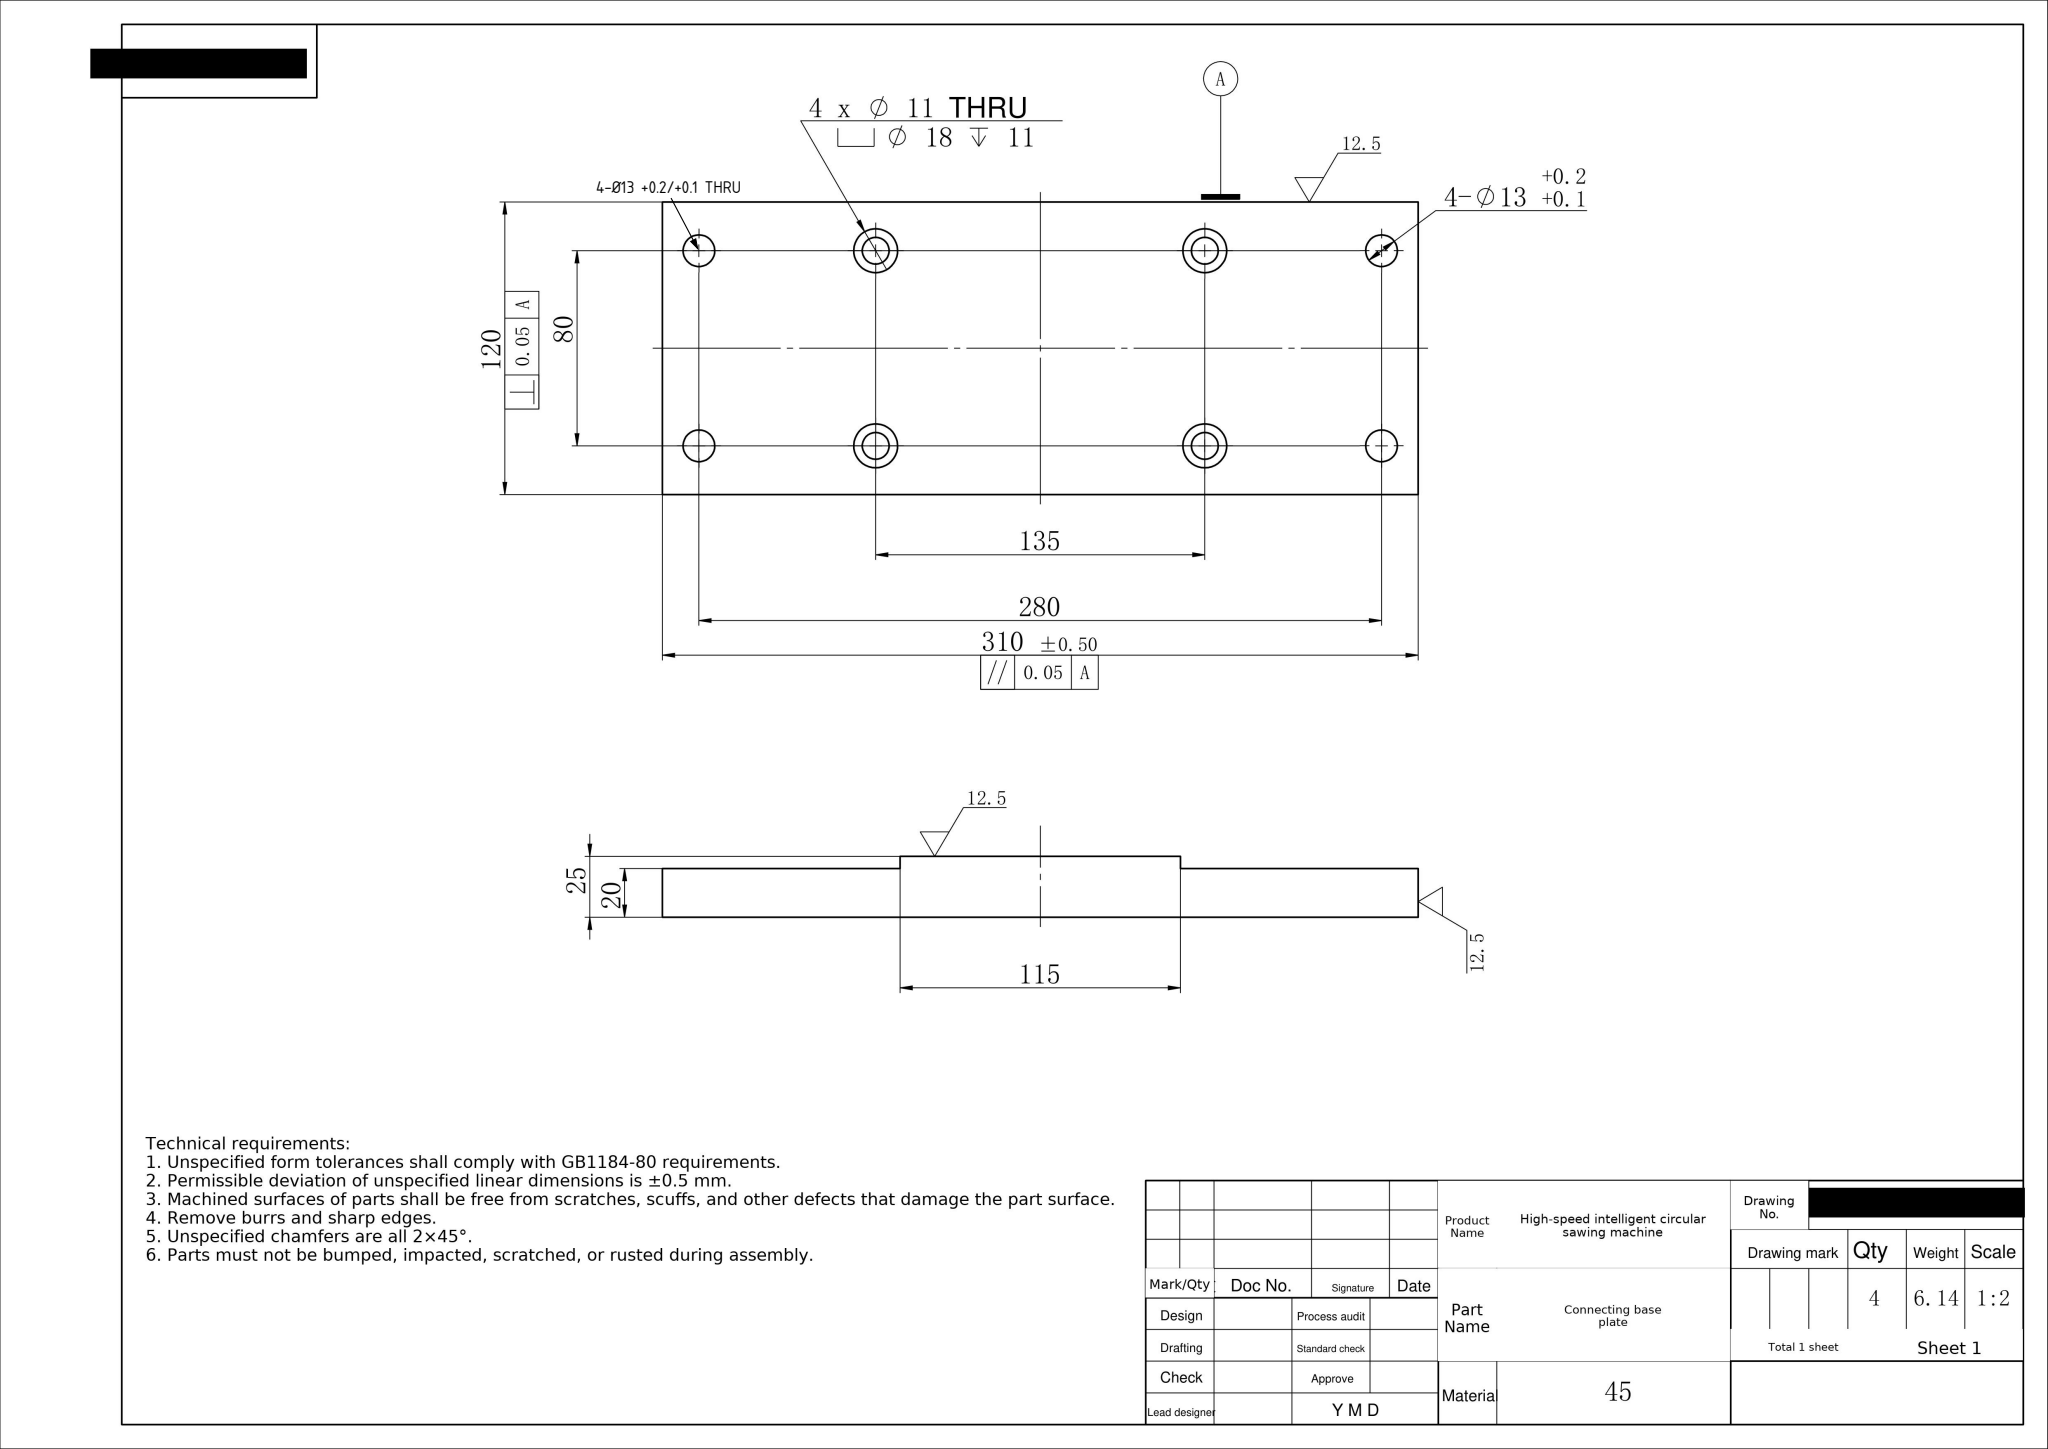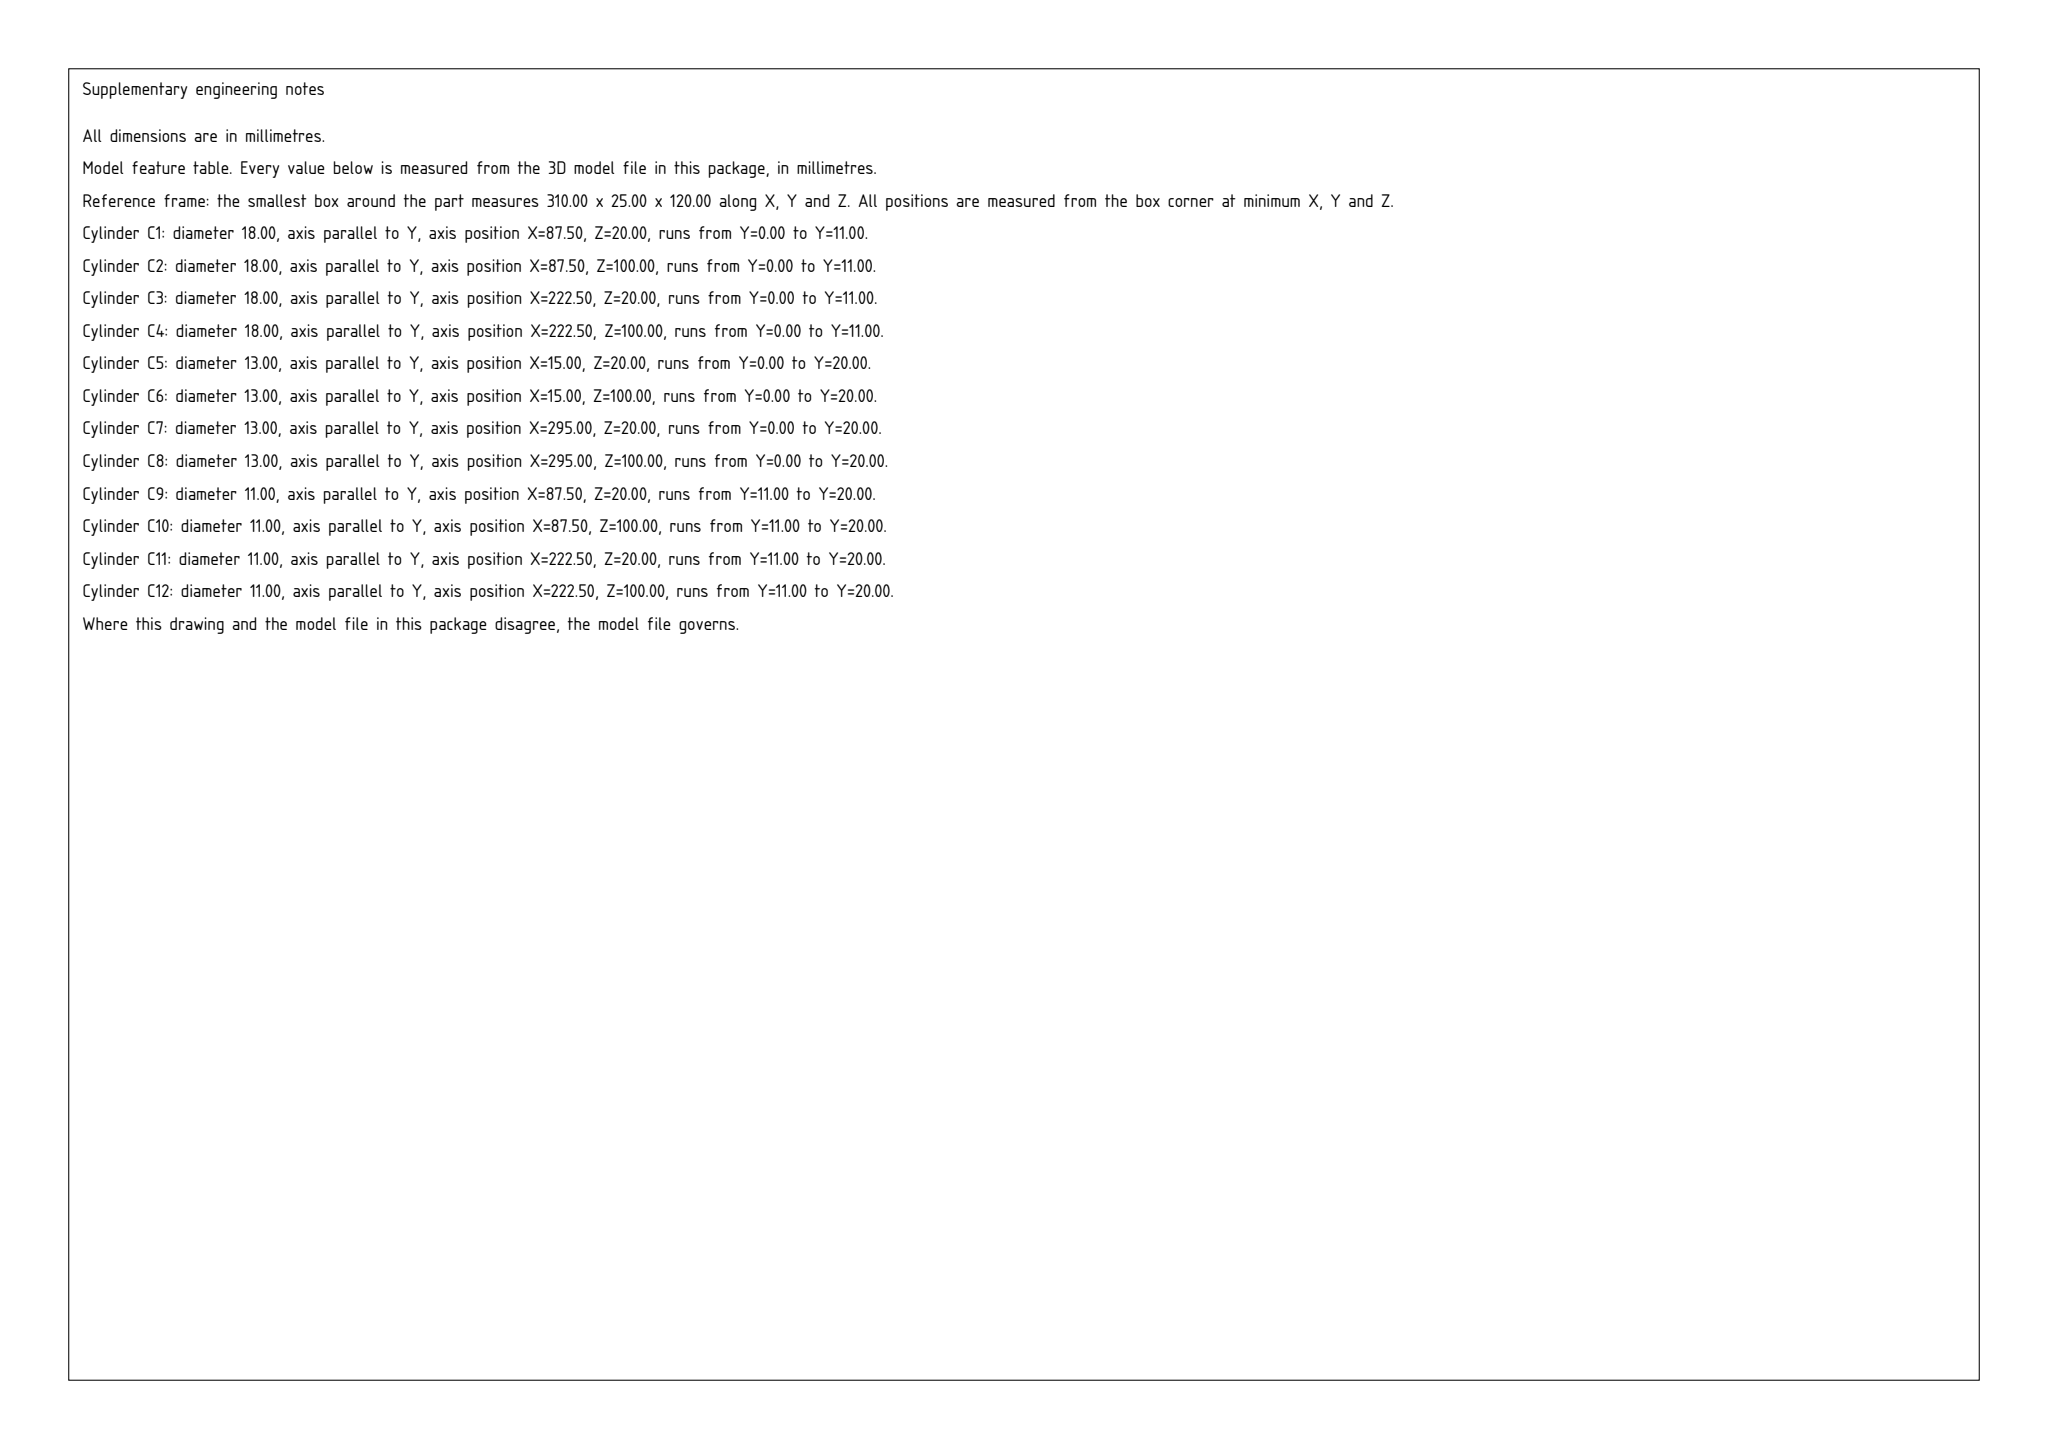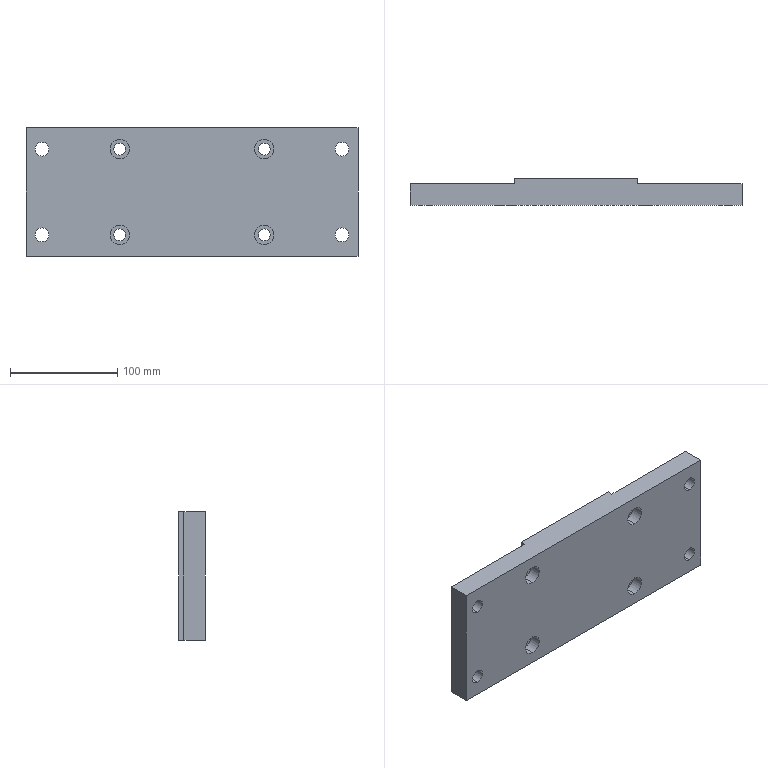Part | SolidWorks | mm | material 45 | 1 solid | 38 faces | box 310 x 25 x 120 mm | volume 787764 mm3 | cylinder 24 | plane 14 | commonest cylinder face diameters 18 x8 11 x8 13 x8
Drawing notes:
4-Ø13 +0.2/+0.1 THRU 20 THK END SECTIONS | from the solid: Ø13 cylinders, axis y, length 20.0 = full 20 mm end-section thickness (y planes 0 and 20)
build123d program:
from build123d import *

# Parameters (mm, degrees)
BOSS_EXTRUDE1_DEPTH                               = 120
F_13_0_13_DIAMETER_HOLE1_D                        = 13
HOLE_SIZE_ACCORDING_TO_HEXAGON_SOCKET_D           = 11
HOLE_SIZE_ACCORDING_TO_HEXAGON_SOCKET_CBORE_D     = 18
HOLE_SIZE_ACCORDING_TO_HEXAGON_SOCKET_CBORE_DEPTH = 11


with BuildPart() as part:
    # Sketch1 → Boss-Extrude1 (new body)
    with BuildSketch(Plane.XY):
        Polygon((0, 25), (0, 0), (155, 0), (155, 20), (57.5, 20), (57.5, 25), align=None)
        Polygon((-155, 20), (-155, 0), (0, 0), (0, 25), (-57.5, 25), (-57.5, 20), align=None)
    extrude(amount=BOSS_EXTRUDE1_DEPTH)

    # 13.0 _13_ Diameter Hole1 (through all)
    with Locations(Plane(origin=(0, 20, 0), x_dir=(1, 0, 0), z_dir=(0, 1, 0))):
        with Locations((140, -20), (140, -100), (-140, -20), (-140, -100)):
            Hole(F_13_0_13_DIAMETER_HOLE1_D / 2)

    # Hole Size _According to_ Hexagon Socket (through all)
    with Locations(Plane(origin=(0, 0, 0), x_dir=(-1, 0, 0), z_dir=(0, -1, 0))):
        with Locations((-67.5, -20), (67.5, -20), (-67.5, -100), (67.5, -100)):
            CounterBoreHole(HOLE_SIZE_ACCORDING_TO_HEXAGON_SOCKET_D / 2, HOLE_SIZE_ACCORDING_TO_HEXAGON_SOCKET_CBORE_D / 2, HOLE_SIZE_ACCORDING_TO_HEXAGON_SOCKET_CBORE_DEPTH)


solid = part.part